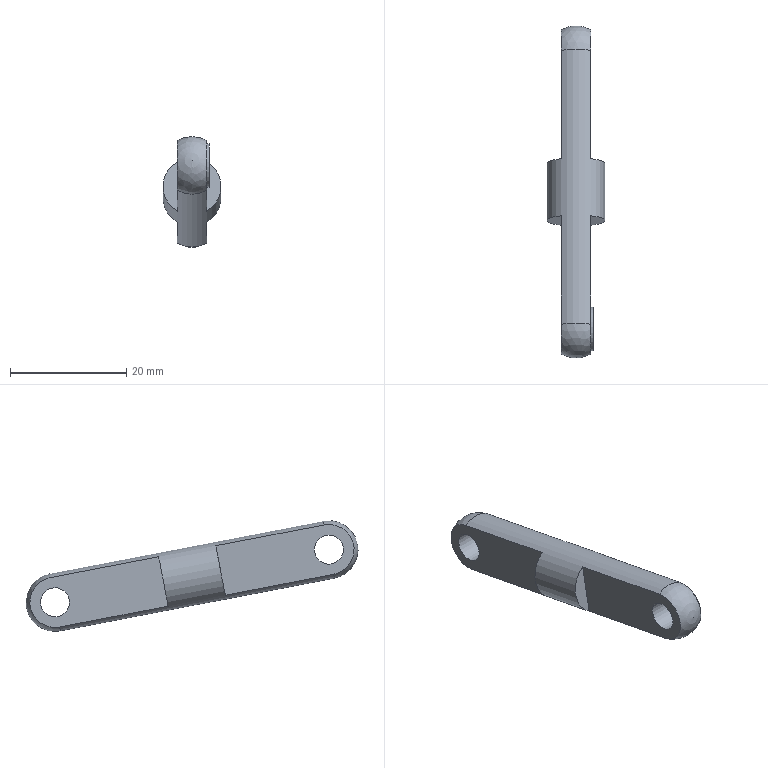Component | NX | CONNECTING_ROD | 1 solid | 15 faces | volume 2779 mm3 | plane 9 | cylinder 4 | sphere 2 | commonest cylinder face diameters 5 x2 10 x1 7.5 x1